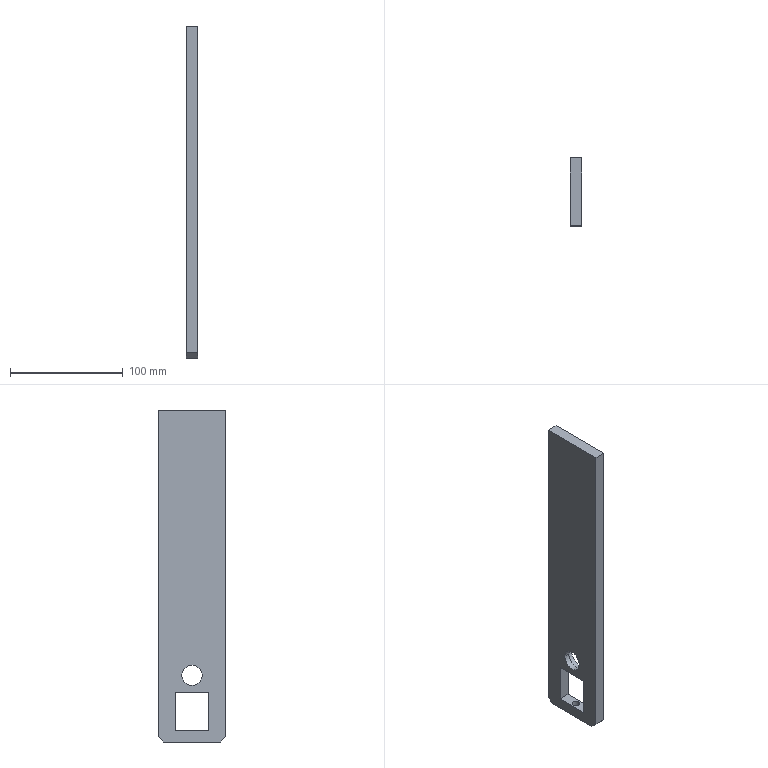Component | SolidWorks | SupportPlate-2 | 1 solid | 25 faces | box 10 x 60 x 294 mm | volume 162382 mm3 | plane 15 | cylinder 10 | commonest cylinder face diameters 8 x4 6.8 x2 18 x2 21 x2
build123d program:
from build123d import *

# Parameters (mm, degrees)
SKETCH1_W             = 60
SKETCH1_H             = 300
BOSS_EXTRUDE1_DEPTH   = 10
SKETCH2_R             = 10.5
CUT_EXTRUDE1_DEPTH    = 5
SKETCH3_R             = 9
CUT_EXTRUDE2_DEPTH    = 306.982
SKETCH4_W             = 30
SKETCH4_H             = 50
CUT_EXTRUDE3_DEPTH    = 307.105
SKETCH5_R             = 4
CUT_EXTRUDE4_DEPTH    = 2
SKETCH6_W             = 30
SKETCH6_H             = 16
BOSS_EXTRUDE2_DEPTH   = 10
SKETCH7_W             = 74.928
SKETCH7_H             = 16.817
CUT_EXTRUDE5_DEPTH    = 307.105
CHAMFER1_SIZE         = 5
M8_TAPPED_HOLE1_D     = 6.8
M8_TAPPED_HOLE1_DEPTH = 19.75
M8_TAPPED_HOLE1_TIP   = 2.043


with BuildPart() as part:
    # Sketch1 → Boss-Extrude1 (new body)
    with BuildSketch(Plane.XY):
        with Locations((30, -150)):
            Rectangle(SKETCH1_W, SKETCH1_H)
    extrude(amount=BOSS_EXTRUDE1_DEPTH)

    # Sketch2 → Cut-Extrude1 (cut)
    with BuildSketch(Plane.XY.offset(10)):
        with Locations((30, -25)):
            Circle(SKETCH2_R)
        with Locations((30, -65)):
            Circle(SKETCH2_R)
    extrude(amount=-CUT_EXTRUDE1_DEPTH, mode=Mode.SUBTRACT)

    # Sketch3 → Cut-Extrude2 (cut, through all)
    with BuildSketch(Plane.XY.offset(5)):
        with Locations((30, -25)):
            Circle(SKETCH3_R)
        with Locations((30, -65)):
            Circle(SKETCH3_R)
    extrude(amount=-CUT_EXTRUDE2_DEPTH, mode=Mode.SUBTRACT)

    # Sketch4 → Cut-Extrude3 (cut, through all)
    with BuildSketch(Plane.XY.offset(10)):
        with Locations((30, -25)):
            Rectangle(SKETCH4_W, SKETCH4_H)
    extrude(amount=-CUT_EXTRUDE3_DEPTH, mode=Mode.SUBTRACT)

    # Sketch5 → Cut-Extrude4 (cut)
    with BuildSketch(Plane(origin=(0, -50, 0), x_dir=(1, 0, 0), z_dir=(0, 1, 0))):
        with Locations(Location((19.5, -5, 0), (0, 0, 270))):
            Circle(SKETCH5_R)
        with Locations(Location((40.5, -5, 0), (0, 0, 270))):
            Circle(SKETCH5_R)
    extrude(amount=-CUT_EXTRUDE4_DEPTH, mode=Mode.SUBTRACT)

    # Sketch6 → Boss-Extrude2 (add)
    with BuildSketch(Plane(origin=(0, 0, 0), x_dir=(-1, 0, 0), z_dir=(0, 0, -1))):
        with Locations((-30, -8)):
            Rectangle(SKETCH6_W, SKETCH6_H)
    extrude(amount=-BOSS_EXTRUDE2_DEPTH)

    # Sketch7 → Cut-Extrude5 (cut, through all)
    with BuildSketch(Plane.XY.offset(10)):
        with Locations((27.689, 2.409)):
            Rectangle(SKETCH7_W, SKETCH7_H)
    extrude(amount=-CUT_EXTRUDE5_DEPTH, mode=Mode.SUBTRACT)

    # Chamfer1
    chamfer1_edges = [part.edges().sort_by_distance(p)[0] for p in [
        (0, -6, 5),
        (60, -6, 5),
    ]]
    chamfer(chamfer1_edges, length=CHAMFER1_SIZE)

    # M8 Tapped Hole1
    with Locations(Plane(origin=(0, -6, 0), x_dir=(1, 0, 0), z_dir=(0, 1, 0))):
        with Locations((30, -5)):
            Hole(M8_TAPPED_HOLE1_D / 2, depth=M8_TAPPED_HOLE1_DEPTH)
            with Locations((0, 0, -(M8_TAPPED_HOLE1_DEPTH + M8_TAPPED_HOLE1_TIP / 2))):  # 118° drill point
                Cone(0, M8_TAPPED_HOLE1_D / 2, M8_TAPPED_HOLE1_TIP, mode=Mode.SUBTRACT)


solid = part.part

# Placed as in the assembly
solid = solid.moved(Location((0, 0, -207.268), (-90, 90, 0)))
STEP:
#1=COLOUR_RGB('',0.7922,0.8196,0.9333);
#2=FILL_AREA_STYLE_COLOUR('',#1);
#3=FILL_AREA_STYLE('',(#2));
#4=SURFACE_STYLE_FILL_AREA(#3);
#5=SURFACE_SIDE_STYLE('',(#4));
#6=SURFACE_STYLE_USAGE(.BOTH.,#5);
#7=PRESENTATION_STYLE_ASSIGNMENT((#6));
#8=CARTESIAN_POINT('',(0.3307,-1.181,-7.53));
#9=VERTEX_POINT('',#8);
#10=CARTESIAN_POINT('',(0.06299,-1.181,-7.53));
#11=VERTEX_POINT('',#10);
#12=CARTESIAN_POINT('',(0.1969,-1.181,-7.53));
#13=DIRECTION('',(0.,0.,1.));
#14=DIRECTION('',(-1.,0.,0.));
#15=AXIS2_PLACEMENT_3D('',#12,#13,#14);
#16=CIRCLE('',#15,0.1339);
#17=EDGE_CURVE('',#9,#11,#16,.T.);
#18=ORIENTED_EDGE('',*,*,#17,.T.);
#19=CARTESIAN_POINT('',(0.06299,-1.181,-7.924));
#20=VERTEX_POINT('',#19);
#21=CARTESIAN_POINT('',(0.06299,-1.181,-7.924));
#22=DIRECTION('',(-0.,-0.,-1.));
#23=VECTOR('',#22,39.37);
#24=LINE('',#21,#23);
#25=EDGE_CURVE('',#11,#20,#24,.T.);
#26=ORIENTED_EDGE('',*,*,#25,.T.);
#27=CARTESIAN_POINT('',(0.3307,-1.181,-7.924));
#28=VERTEX_POINT('',#27);
#29=CARTESIAN_POINT('',(0.1969,-1.181,-7.924));
#30=DIRECTION('',(-0.,-0.,-1.));
#31=DIRECTION('',(1.,0.,0.));
#32=AXIS2_PLACEMENT_3D('',#29,#30,#31);
#33=CIRCLE('',#32,0.1339);
#34=EDGE_CURVE('',#20,#28,#33,.T.);
#35=ORIENTED_EDGE('',*,*,#34,.T.);
#36=CARTESIAN_POINT('',(0.3307,-1.181,-7.924));
#37=DIRECTION('',(-0.,-0.,-1.));
#38=VECTOR('',#37,39.37);
#39=LINE('',#36,#38);
#40=EDGE_CURVE('',#9,#28,#39,.T.);
#41=ORIENTED_EDGE('',*,*,#40,.F.);
#42=EDGE_LOOP('',(#18,#26,#35,#41));
#43=FACE_OUTER_BOUND('',#42,.T.);
#44=CARTESIAN_POINT('',(0.1969,-1.181,-7.924));
#45=DIRECTION('',(-0.,-0.,-1.));
#46=DIRECTION('',(1.,0.,0.));
#47=AXIS2_PLACEMENT_3D('',#44,#45,#46);
#48=CYLINDRICAL_SURFACE('',#47,0.1339);
#49=ADVANCED_FACE('',(#43),#48,.F.);
#50=CARTESIAN_POINT('',(0.03937,-1.594,-6.113));
#51=VERTEX_POINT('',#50);
#52=CARTESIAN_POINT('',(0.3543,-1.594,-6.113));
#53=VERTEX_POINT('',#52);
#54=CARTESIAN_POINT('',(0.1969,-1.594,-6.113));
#55=DIRECTION('',(-0.,-0.,-1.));
#56=DIRECTION('',(1.,0.,0.));
#57=AXIS2_PLACEMENT_3D('',#54,#55,#56);
#58=CIRCLE('',#57,0.1575);
#59=EDGE_CURVE('',#51,#53,#58,.T.);
#60=ORIENTED_EDGE('',*,*,#59,.F.);
#61=CARTESIAN_POINT('',(0.03937,-1.594,-6.192));
#62=VERTEX_POINT('',#61);
#63=CARTESIAN_POINT('',(0.03937,-1.594,-6.113));
#64=DIRECTION('',(-0.,-0.,-1.));
#65=VECTOR('',#64,39.37);
#66=LINE('',#63,#65);
#67=EDGE_CURVE('',#51,#62,#66,.T.);
#68=ORIENTED_EDGE('',*,*,#67,.T.);
#69=CARTESIAN_POINT('',(0.3543,-1.594,-6.192));
#70=VERTEX_POINT('',#69);
#71=CARTESIAN_POINT('',(0.1969,-1.594,-6.192));
#72=DIRECTION('',(-0.,-0.,-1.));
#73=DIRECTION('',(1.,0.,0.));
#74=AXIS2_PLACEMENT_3D('',#71,#72,#73);
#75=CIRCLE('',#74,0.1575);
#76=EDGE_CURVE('',#62,#70,#75,.T.);
#77=ORIENTED_EDGE('',*,*,#76,.T.);
#78=CARTESIAN_POINT('',(0.3543,-1.594,-6.113));
#79=DIRECTION('',(-0.,-0.,-1.));
#80=VECTOR('',#79,39.37);
#81=LINE('',#78,#80);
#82=EDGE_CURVE('',#53,#70,#81,.T.);
#83=ORIENTED_EDGE('',*,*,#82,.F.);
#84=EDGE_LOOP('',(#60,#68,#77,#83));
#85=FACE_OUTER_BOUND('',#84,.T.);
#86=CARTESIAN_POINT('',(0.1969,-1.594,-6.113));
#87=DIRECTION('',(-0.,-0.,-1.));
#88=DIRECTION('',(1.,0.,0.));
#89=AXIS2_PLACEMENT_3D('',#86,#87,#88);
#90=CYLINDRICAL_SURFACE('',#89,0.1575);
#91=ADVANCED_FACE('',(#85),#90,.F.);
#92=CARTESIAN_POINT('',(0.03937,-0.7677,-6.113));
#93=VERTEX_POINT('',#92);
#94=CARTESIAN_POINT('',(0.3543,-0.7677,-6.113));
#95=VERTEX_POINT('',#94);
#96=CARTESIAN_POINT('',(0.1969,-0.7677,-6.113));
#97=DIRECTION('',(-0.,-0.,-1.));
#98=DIRECTION('',(1.,0.,0.));
#99=AXIS2_PLACEMENT_3D('',#96,#97,#98);
#100=CIRCLE('',#99,0.1575);
#101=EDGE_CURVE('',#93,#95,#100,.T.);
#102=ORIENTED_EDGE('',*,*,#101,.F.);
#103=CARTESIAN_POINT('',(0.03937,-0.7677,-6.192));
#104=VERTEX_POINT('',#103);
#105=CARTESIAN_POINT('',(0.03937,-0.7677,-6.113));
#106=DIRECTION('',(-0.,-0.,-1.));
#107=VECTOR('',#106,39.37);
#108=LINE('',#105,#107);
#109=EDGE_CURVE('',#93,#104,#108,.T.);
#110=ORIENTED_EDGE('',*,*,#109,.T.);
#111=CARTESIAN_POINT('',(0.3543,-0.7677,-6.192));
#112=VERTEX_POINT('',#111);
#113=CARTESIAN_POINT('',(0.1969,-0.7677,-6.192));
#114=DIRECTION('',(-0.,-0.,-1.));
#115=DIRECTION('',(1.,0.,0.));
#116=AXIS2_PLACEMENT_3D('',#113,#114,#115);
#117=CIRCLE('',#116,0.1575);
#118=EDGE_CURVE('',#104,#112,#117,.T.);
#119=ORIENTED_EDGE('',*,*,#118,.T.);
#120=CARTESIAN_POINT('',(0.3543,-0.7677,-6.113));
#121=DIRECTION('',(-0.,-0.,-1.));
#122=VECTOR('',#121,39.37);
#123=LINE('',#120,#122);
#124=EDGE_CURVE('',#95,#112,#123,.T.);
#125=ORIENTED_EDGE('',*,*,#124,.F.);
#126=EDGE_LOOP('',(#102,#110,#119,#125));
#127=FACE_OUTER_BOUND('',#126,.T.);
#128=CARTESIAN_POINT('',(0.1969,-0.7677,-6.113));
#129=DIRECTION('',(-0.,-0.,-1.));
#130=DIRECTION('',(1.,0.,0.));
#131=AXIS2_PLACEMENT_3D('',#128,#129,#130);
#132=CYLINDRICAL_SURFACE('',#131,0.1575);
#133=ADVANCED_FACE('',(#127),#132,.F.);
#134=CARTESIAN_POINT('',(-0.,-0.8268,-5.601));
#135=VERTEX_POINT('',#134);
#136=CARTESIAN_POINT('',(-0.,-1.535,-5.601));
#137=VERTEX_POINT('',#136);
#138=CARTESIAN_POINT('',(-0.,-1.181,-5.601));
#139=DIRECTION('',(1.,0.,-0.));
#140=DIRECTION('',(0.,-1.,0.));
#141=AXIS2_PLACEMENT_3D('',#138,#139,#140);
#142=CIRCLE('',#141,0.3543);
#143=EDGE_CURVE('',#135,#137,#142,.T.);
#144=ORIENTED_EDGE('',*,*,#143,.F.);
#145=CARTESIAN_POINT('',(0.1969,-0.8268,-5.601));
#146=VERTEX_POINT('',#145);
#147=CARTESIAN_POINT('',(-0.,-0.8268,-5.601));
#148=DIRECTION('',(1.,0.,-0.));
#149=VECTOR('',#148,39.37);
#150=LINE('',#147,#149);
#151=EDGE_CURVE('',#135,#146,#150,.T.);
#152=ORIENTED_EDGE('',*,*,#151,.T.);
#153=CARTESIAN_POINT('',(0.1969,-1.535,-5.601));
#154=VERTEX_POINT('',#153);
#155=CARTESIAN_POINT('',(0.1969,-1.181,-5.601));
#156=DIRECTION('',(1.,0.,-0.));
#157=DIRECTION('',(0.,-1.,0.));
#158=AXIS2_PLACEMENT_3D('',#155,#156,#157);
#159=CIRCLE('',#158,0.3543);
#160=EDGE_CURVE('',#146,#154,#159,.T.);
#161=ORIENTED_EDGE('',*,*,#160,.T.);
#162=CARTESIAN_POINT('',(-0.,-1.535,-5.601));
#163=DIRECTION('',(1.,0.,-0.));
#164=VECTOR('',#163,39.37);
#165=LINE('',#162,#164);
#166=EDGE_CURVE('',#137,#154,#165,.T.);
#167=ORIENTED_EDGE('',*,*,#166,.F.);
#168=EDGE_LOOP('',(#144,#152,#161,#167));
#169=FACE_OUTER_BOUND('',#168,.T.);
#170=CARTESIAN_POINT('',(-0.,-1.181,-5.601));
#171=DIRECTION('',(1.,0.,-0.));
#172=DIRECTION('',(0.,-1.,0.));
#173=AXIS2_PLACEMENT_3D('',#170,#171,#172);
#174=CYLINDRICAL_SURFACE('',#173,0.3543);
#175=ADVANCED_FACE('',(#169),#174,.F.);
#176=CARTESIAN_POINT('',(0.1969,-0.7677,-5.601));
#177=VERTEX_POINT('',#176);
#178=CARTESIAN_POINT('',(0.1969,-1.594,-5.601));
#179=VERTEX_POINT('',#178);
#180=CARTESIAN_POINT('',(0.1969,-1.181,-5.601));
#181=DIRECTION('',(1.,0.,-0.));
#182=DIRECTION('',(0.,-1.,0.));
#183=AXIS2_PLACEMENT_3D('',#180,#181,#182);
#184=CIRCLE('',#183,0.4134);
#185=EDGE_CURVE('',#177,#179,#184,.T.);
#186=ORIENTED_EDGE('',*,*,#185,.F.);
#187=CARTESIAN_POINT('',(0.3937,-0.7677,-5.601));
#188=VERTEX_POINT('',#187);
#189=CARTESIAN_POINT('',(0.1969,-0.7677,-5.601));
#190=DIRECTION('',(1.,0.,-0.));
#191=VECTOR('',#190,39.37);
#192=LINE('',#189,#191);
#193=EDGE_CURVE('',#177,#188,#192,.T.);
#194=ORIENTED_EDGE('',*,*,#193,.T.);
#195=CARTESIAN_POINT('',(0.3937,-1.594,-5.601));
#196=VERTEX_POINT('',#195);
#197=CARTESIAN_POINT('',(0.3937,-1.181,-5.601));
#198=DIRECTION('',(1.,0.,-0.));
#199=DIRECTION('',(0.,-1.,0.));
#200=AXIS2_PLACEMENT_3D('',#197,#198,#199);
#201=CIRCLE('',#200,0.4134);
#202=EDGE_CURVE('',#188,#196,#201,.T.);
#203=ORIENTED_EDGE('',*,*,#202,.T.);
#204=CARTESIAN_POINT('',(0.1969,-1.594,-5.601));
#205=DIRECTION('',(1.,0.,-0.));
#206=VECTOR('',#205,39.37);
#207=LINE('',#204,#206);
#208=EDGE_CURVE('',#179,#196,#207,.T.);
#209=ORIENTED_EDGE('',*,*,#208,.F.);
#210=EDGE_LOOP('',(#186,#194,#203,#209));
#211=FACE_OUTER_BOUND('',#210,.T.);
#212=CARTESIAN_POINT('',(0.1969,-1.181,-5.601));
#213=DIRECTION('',(1.,0.,-0.));
#214=DIRECTION('',(0.,-1.,0.));
#215=AXIS2_PLACEMENT_3D('',#212,#213,#214);
#216=CYLINDRICAL_SURFACE('',#215,0.4134);
#217=ADVANCED_FACE('',(#211),#216,.F.);
#218=CARTESIAN_POINT('',(0.3937,-0.,-7.727));
#219=VERTEX_POINT('',#218);
#220=CARTESIAN_POINT('',(0.3937,-0.,3.651));
#221=VERTEX_POINT('',#220);
#222=CARTESIAN_POINT('',(0.3937,0.,-8.16));
#223=DIRECTION('',(0.,-0.,1.));
#224=VECTOR('',#223,39.37);
#225=LINE('',#222,#224);
#226=EDGE_CURVE('',#219,#221,#225,.T.);
#227=ORIENTED_EDGE('',*,*,#226,.F.);
#228=CARTESIAN_POINT('',(-0.,-0.,-7.727));
#229=VERTEX_POINT('',#228);
#230=CARTESIAN_POINT('',(0.3937,-0.,-7.727));
#231=DIRECTION('',(-1.,-0.,0.));
#232=VECTOR('',#231,39.37);
#233=LINE('',#230,#232);
#234=EDGE_CURVE('',#219,#229,#233,.T.);
#235=ORIENTED_EDGE('',*,*,#234,.T.);
#236=CARTESIAN_POINT('',(-0.,-0.,3.651));
#237=VERTEX_POINT('',#236);
#238=CARTESIAN_POINT('',(-0.,0.,-8.16));
#239=DIRECTION('',(0.,-0.,1.));
#240=VECTOR('',#239,39.37);
#241=LINE('',#238,#240);
#242=EDGE_CURVE('',#229,#237,#241,.T.);
#243=ORIENTED_EDGE('',*,*,#242,.T.);
#244=CARTESIAN_POINT('',(0.3937,-0.,3.651));
#245=DIRECTION('',(-1.,-0.,0.));
#246=VECTOR('',#245,39.37);
#247=LINE('',#244,#246);
#248=EDGE_CURVE('',#221,#237,#247,.T.);
#249=ORIENTED_EDGE('',*,*,#248,.F.);
#250=EDGE_LOOP('',(#227,#235,#243,#249));
#251=FACE_OUTER_BOUND('',#250,.T.);
#252=CARTESIAN_POINT('',(0.3937,0.,-8.16));
#253=DIRECTION('',(0.,-1.,-0.));
#254=DIRECTION('',(-0.,0.,-1.));
#255=AXIS2_PLACEMENT_3D('',#252,#253,#254);
#256=PLANE('',#255);
#257=ADVANCED_FACE('',(#251),#256,.F.);
#258=CARTESIAN_POINT('',(-0.,-2.362,3.651));
#259=VERTEX_POINT('',#258);
#260=CARTESIAN_POINT('',(-0.,-0.,3.651));
#261=DIRECTION('',(0.,-1.,0.));
#262=VECTOR('',#261,39.37);
#263=LINE('',#260,#262);
#264=EDGE_CURVE('',#237,#259,#263,.T.);
#265=ORIENTED_EDGE('',*,*,#264,.T.);
#266=CARTESIAN_POINT('',(0.3937,-2.362,3.651));
#267=VERTEX_POINT('',#266);
#268=CARTESIAN_POINT('',(0.3937,-2.362,3.651));
#269=DIRECTION('',(-1.,-0.,0.));
#270=VECTOR('',#269,39.37);
#271=LINE('',#268,#270);
#272=EDGE_CURVE('',#267,#259,#271,.T.);
#273=ORIENTED_EDGE('',*,*,#272,.F.);
#274=CARTESIAN_POINT('',(0.3937,-0.,3.651));
#275=DIRECTION('',(0.,-1.,0.));
#276=VECTOR('',#275,39.37);
#277=LINE('',#274,#276);
#278=EDGE_CURVE('',#221,#267,#277,.T.);
#279=ORIENTED_EDGE('',*,*,#278,.F.);
#280=ORIENTED_EDGE('',*,*,#248,.T.);
#281=EDGE_LOOP('',(#265,#273,#279,#280));
#282=FACE_OUTER_BOUND('',#281,.T.);
#283=CARTESIAN_POINT('',(0.3937,-0.,3.651));
#284=DIRECTION('',(-0.,-0.,-1.));
#285=DIRECTION('',(1.,0.,-0.));
#286=AXIS2_PLACEMENT_3D('',#283,#284,#285);
#287=PLANE('',#286);
#288=ADVANCED_FACE('',(#282),#287,.F.);
#289=CARTESIAN_POINT('',(-0.,-2.362,-7.727));
#290=VERTEX_POINT('',#289);
#291=CARTESIAN_POINT('',(-0.,-2.362,-8.16));
#292=DIRECTION('',(-0.,0.,-1.));
#293=VECTOR('',#292,39.37);
#294=LINE('',#291,#293);
#295=EDGE_CURVE('',#259,#290,#294,.T.);
#296=ORIENTED_EDGE('',*,*,#295,.T.);
#297=CARTESIAN_POINT('',(0.3937,-2.362,-7.727));
#298=VERTEX_POINT('',#297);
#299=CARTESIAN_POINT('',(0.3937,-2.362,-7.727));
#300=DIRECTION('',(1.,0.,-0.));
#301=VECTOR('',#300,39.37);
#302=LINE('',#299,#301);
#303=EDGE_CURVE('',#290,#298,#302,.T.);
#304=ORIENTED_EDGE('',*,*,#303,.T.);
#305=CARTESIAN_POINT('',(0.3937,-2.362,-8.16));
#306=DIRECTION('',(-0.,0.,-1.));
#307=VECTOR('',#306,39.37);
#308=LINE('',#305,#307);
#309=EDGE_CURVE('',#267,#298,#308,.T.);
#310=ORIENTED_EDGE('',*,*,#309,.F.);
#311=ORIENTED_EDGE('',*,*,#272,.T.);
#312=EDGE_LOOP('',(#296,#304,#310,#311));
#313=FACE_OUTER_BOUND('',#312,.T.);
#314=CARTESIAN_POINT('',(0.3937,-2.362,-8.16));
#315=DIRECTION('',(-0.,1.,0.));
#316=DIRECTION('',(0.,-0.,1.));
#317=AXIS2_PLACEMENT_3D('',#314,#315,#316);
#318=PLANE('',#317);
#319=ADVANCED_FACE('',(#313),#318,.F.);
#320=CARTESIAN_POINT('',(0.3937,-0.1969,-7.924));
#321=VERTEX_POINT('',#320);
#322=CARTESIAN_POINT('',(0.3937,-2.165,-7.924));
#323=VERTEX_POINT('',#322);
#324=CARTESIAN_POINT('',(0.3937,0.3848,-7.924));
#325=DIRECTION('',(0.,-1.,0.));
#326=VECTOR('',#325,39.37);
#327=LINE('',#324,#326);
#328=EDGE_CURVE('',#321,#323,#327,.T.);
#329=ORIENTED_EDGE('',*,*,#328,.F.);
#330=CARTESIAN_POINT('',(0.3937,-0.2165,-7.944));
#331=DIRECTION('',(0.,0.7071,0.7071));
#332=VECTOR('',#331,39.37);
#333=LINE('',#330,#332);
#334=EDGE_CURVE('',#321,#219,#333,.T.);
#335=ORIENTED_EDGE('',*,*,#334,.T.);
#336=ORIENTED_EDGE('',*,*,#226,.T.);
#337=ORIENTED_EDGE('',*,*,#278,.T.);
#338=ORIENTED_EDGE('',*,*,#309,.T.);
#339=CARTESIAN_POINT('',(0.3937,-0.9646,-9.125));
#340=DIRECTION('',(-0.,0.7071,-0.7071));
#341=VECTOR('',#340,39.37);
#342=LINE('',#339,#341);
#343=EDGE_CURVE('',#298,#323,#342,.T.);
#344=ORIENTED_EDGE('',*,*,#343,.T.);
#345=EDGE_LOOP('',(#329,#335,#336,#337,#338,#344));
#346=FACE_OUTER_BOUND('',#345,.T.);
#347=CARTESIAN_POINT('',(0.3937,-0.5906,-7.53));
#348=VERTEX_POINT('',#347);
#349=CARTESIAN_POINT('',(0.3937,-0.5906,-6.192));
#350=VERTEX_POINT('',#349);
#351=CARTESIAN_POINT('',(0.3937,-0.5906,-8.16));
#352=DIRECTION('',(0.,0.,1.));
#353=VECTOR('',#352,39.37);
#354=LINE('',#351,#353);
#355=EDGE_CURVE('',#348,#350,#354,.T.);
#356=ORIENTED_EDGE('',*,*,#355,.F.);
#357=CARTESIAN_POINT('',(0.3937,-1.772,-7.53));
#358=VERTEX_POINT('',#357);
#359=CARTESIAN_POINT('',(0.3937,-1.772,-7.53));
#360=DIRECTION('',(-0.,1.,-0.));
#361=VECTOR('',#360,39.37);
#362=LINE('',#359,#361);
#363=EDGE_CURVE('',#358,#348,#362,.T.);
#364=ORIENTED_EDGE('',*,*,#363,.F.);
#365=CARTESIAN_POINT('',(0.3937,-1.772,-6.192));
#366=VERTEX_POINT('',#365);
#367=CARTESIAN_POINT('',(0.3937,-1.772,-8.16));
#368=DIRECTION('',(-0.,-0.,-1.));
#369=VECTOR('',#368,39.37);
#370=LINE('',#367,#369);
#371=EDGE_CURVE('',#366,#358,#370,.T.);
#372=ORIENTED_EDGE('',*,*,#371,.F.);
#373=CARTESIAN_POINT('',(0.3937,-0.5906,-6.192));
#374=DIRECTION('',(0.,-1.,0.));
#375=VECTOR('',#374,39.37);
#376=LINE('',#373,#375);
#377=EDGE_CURVE('',#350,#366,#376,.T.);
#378=ORIENTED_EDGE('',*,*,#377,.F.);
#379=EDGE_LOOP('',(#356,#364,#372,#378));
#380=FACE_BOUND('',#379,.T.);
#381=CARTESIAN_POINT('',(0.3937,-1.181,-5.601));
#382=DIRECTION('',(1.,0.,-0.));
#383=DIRECTION('',(0.,-1.,0.));
#384=AXIS2_PLACEMENT_3D('',#381,#382,#383);
#385=CIRCLE('',#384,0.4134);
#386=EDGE_CURVE('',#196,#188,#385,.T.);
#387=ORIENTED_EDGE('',*,*,#386,.F.);
#388=ORIENTED_EDGE('',*,*,#202,.F.);
#389=EDGE_LOOP('',(#387,#388));
#390=FACE_BOUND('',#389,.T.);
#391=CARTESIAN_POINT('',(0.3937,0.,-8.16));
#392=DIRECTION('',(1.,0.,-0.));
#393=DIRECTION('',(0.,-1.,0.));
#394=AXIS2_PLACEMENT_3D('',#391,#392,#393);
#395=PLANE('',#394);
#396=ADVANCED_FACE('',(#346,#380,#390),#395,.T.);
#397=CARTESIAN_POINT('',(-0.,-1.772,-7.53));
#398=VERTEX_POINT('',#397);
#399=CARTESIAN_POINT('',(-0.,-0.5906,-7.53));
#400=VERTEX_POINT('',#399);
#401=CARTESIAN_POINT('',(-0.,-1.772,-7.53));
#402=DIRECTION('',(-0.,1.,-0.));
#403=VECTOR('',#402,39.37);
#404=LINE('',#401,#403);
#405=EDGE_CURVE('',#398,#400,#404,.T.);
#406=ORIENTED_EDGE('',*,*,#405,.T.);
#407=CARTESIAN_POINT('',(-0.,-0.5906,-6.192));
#408=VERTEX_POINT('',#407);
#409=CARTESIAN_POINT('',(-0.,-0.5906,-8.16));
#410=DIRECTION('',(0.,0.,1.));
#411=VECTOR('',#410,39.37);
#412=LINE('',#409,#411);
#413=EDGE_CURVE('',#400,#408,#412,.T.);
#414=ORIENTED_EDGE('',*,*,#413,.T.);
#415=CARTESIAN_POINT('',(-0.,-1.772,-6.192));
#416=VERTEX_POINT('',#415);
#417=CARTESIAN_POINT('',(-0.,-0.5906,-6.192));
#418=DIRECTION('',(0.,-1.,0.));
#419=VECTOR('',#418,39.37);
#420=LINE('',#417,#419);
#421=EDGE_CURVE('',#408,#416,#420,.T.);
#422=ORIENTED_EDGE('',*,*,#421,.T.);
#423=CARTESIAN_POINT('',(-0.,-1.772,-8.16));
#424=DIRECTION('',(-0.,-0.,-1.));
#425=VECTOR('',#424,39.37);
#426=LINE('',#423,#425);
#427=EDGE_CURVE('',#416,#398,#426,.T.);
#428=ORIENTED_EDGE('',*,*,#427,.T.);
#429=EDGE_LOOP('',(#406,#414,#422,#428));
#430=FACE_BOUND('',#429,.T.);
#431=ORIENTED_EDGE('',*,*,#242,.F.);
#432=CARTESIAN_POINT('',(-0.,-0.1969,-7.924));
#433=VERTEX_POINT('',#432);
#434=CARTESIAN_POINT('',(-0.,-0.,-7.727));
#435=DIRECTION('',(-0.,-0.7071,-0.7071));
#436=VECTOR('',#435,39.37);
#437=LINE('',#434,#436);
#438=EDGE_CURVE('',#229,#433,#437,.T.);
#439=ORIENTED_EDGE('',*,*,#438,.T.);
#440=CARTESIAN_POINT('',(-0.,-2.165,-7.924));
#441=VERTEX_POINT('',#440);
#442=CARTESIAN_POINT('',(-0.,0.,-7.924));
#443=DIRECTION('',(0.,-1.,0.));
#444=VECTOR('',#443,39.37);
#445=LINE('',#442,#444);
#446=EDGE_CURVE('',#433,#441,#445,.T.);
#447=ORIENTED_EDGE('',*,*,#446,.T.);
#448=CARTESIAN_POINT('',(-0.,-2.362,-7.727));
#449=DIRECTION('',(0.,-0.7071,0.7071));
#450=VECTOR('',#449,39.37);
#451=LINE('',#448,#450);
#452=EDGE_CURVE('',#441,#290,#451,.T.);
#453=ORIENTED_EDGE('',*,*,#452,.T.);
#454=ORIENTED_EDGE('',*,*,#295,.F.);
#455=ORIENTED_EDGE('',*,*,#264,.F.);
#456=EDGE_LOOP('',(#431,#439,#447,#453,#454,#455));
#457=FACE_OUTER_BOUND('',#456,.T.);
#458=CARTESIAN_POINT('',(-0.,-1.181,-5.601));
#459=DIRECTION('',(1.,0.,-0.));
#460=DIRECTION('',(0.,-1.,0.));
#461=AXIS2_PLACEMENT_3D('',#458,#459,#460);
#462=CIRCLE('',#461,0.3543);
#463=EDGE_CURVE('',#137,#135,#462,.T.);
#464=ORIENTED_EDGE('',*,*,#463,.T.);
#465=ORIENTED_EDGE('',*,*,#143,.T.);
#466=EDGE_LOOP('',(#464,#465));
#467=FACE_BOUND('',#466,.T.);
#468=CARTESIAN_POINT('',(-0.,0.,-8.16));
#469=DIRECTION('',(1.,0.,-0.));
#470=DIRECTION('',(0.,-1.,0.));
#471=AXIS2_PLACEMENT_3D('',#468,#469,#470);
#472=PLANE('',#471);
#473=ADVANCED_FACE('',(#430,#457,#467),#472,.F.);
#474=ORIENTED_EDGE('',*,*,#193,.F.);
#475=CARTESIAN_POINT('',(0.1969,-1.181,-5.601));
#476=DIRECTION('',(1.,0.,-0.));
#477=DIRECTION('',(0.,-1.,0.));
#478=AXIS2_PLACEMENT_3D('',#475,#476,#477);
#479=CIRCLE('',#478,0.4134);
#480=EDGE_CURVE('',#179,#177,#479,.T.);
#481=ORIENTED_EDGE('',*,*,#480,.F.);
#482=ORIENTED_EDGE('',*,*,#208,.T.);
#483=ORIENTED_EDGE('',*,*,#386,.T.);
#484=EDGE_LOOP('',(#474,#481,#482,#483));
#485=FACE_OUTER_BOUND('',#484,.T.);
#486=CARTESIAN_POINT('',(0.1969,-1.181,-5.601));
#487=DIRECTION('',(1.,0.,-0.));
#488=DIRECTION('',(0.,-1.,0.));
#489=AXIS2_PLACEMENT_3D('',#486,#487,#488);
#490=CYLINDRICAL_SURFACE('',#489,0.4134);
#491=ADVANCED_FACE('',(#485),#490,.F.);
#492=CARTESIAN_POINT('',(0.1969,-1.181,-5.601));
#493=DIRECTION('',(1.,0.,-0.));
#494=DIRECTION('',(0.,-1.,0.));
#495=AXIS2_PLACEMENT_3D('',#492,#493,#494);
#496=CIRCLE('',#495,0.3543);
#497=EDGE_CURVE('',#154,#146,#496,.T.);
#498=ORIENTED_EDGE('',*,*,#497,.F.);
#499=ORIENTED_EDGE('',*,*,#160,.F.);
#500=EDGE_LOOP('',(#498,#499));
#501=FACE_BOUND('',#500,.T.);
#502=ORIENTED_EDGE('',*,*,#480,.T.);
#503=ORIENTED_EDGE('',*,*,#185,.T.);
#504=EDGE_LOOP('',(#502,#503));
#505=FACE_OUTER_BOUND('',#504,.T.);
#506=CARTESIAN_POINT('',(0.1969,-1.181,-5.601));
#507=DIRECTION('',(1.,0.,-0.));
#508=DIRECTION('',(0.,-1.,0.));
#509=AXIS2_PLACEMENT_3D('',#506,#507,#508);
#510=PLANE('',#509);
#511=ADVANCED_FACE('',(#501,#505),#510,.T.);
#512=ORIENTED_EDGE('',*,*,#151,.F.);
#513=ORIENTED_EDGE('',*,*,#463,.F.);
#514=ORIENTED_EDGE('',*,*,#166,.T.);
#515=ORIENTED_EDGE('',*,*,#497,.T.);
#516=EDGE_LOOP('',(#512,#513,#514,#515));
#517=FACE_OUTER_BOUND('',#516,.T.);
#518=CARTESIAN_POINT('',(-0.,-1.181,-5.601));
#519=DIRECTION('',(1.,0.,-0.));
#520=DIRECTION('',(0.,-1.,0.));
#521=AXIS2_PLACEMENT_3D('',#518,#519,#520);
#522=CYLINDRICAL_SURFACE('',#521,0.3543);
#523=ADVANCED_FACE('',(#517),#522,.F.);
#524=ORIENTED_EDGE('',*,*,#413,.F.);
#525=CARTESIAN_POINT('',(1.732,-0.5906,-7.53));
#526=DIRECTION('',(-1.,-0.,0.));
#527=VECTOR('',#526,39.37);
#528=LINE('',#525,#527);
#529=EDGE_CURVE('',#348,#400,#528,.T.);
#530=ORIENTED_EDGE('',*,*,#529,.F.);
#531=ORIENTED_EDGE('',*,*,#355,.T.);
#532=CARTESIAN_POINT('',(-0.,-0.5906,-6.192));
#533=DIRECTION('',(1.,0.,-0.));
#534=VECTOR('',#533,39.37);
#535=LINE('',#532,#534);
#536=EDGE_CURVE('',#408,#350,#535,.T.);
#537=ORIENTED_EDGE('',*,*,#536,.F.);
#538=EDGE_LOOP('',(#524,#530,#531,#537));
#539=FACE_OUTER_BOUND('',#538,.T.);
#540=CARTESIAN_POINT('',(-0.,-0.5906,-8.16));
#541=DIRECTION('',(-0.,1.,-0.));
#542=DIRECTION('',(0.,0.,1.));
#543=AXIS2_PLACEMENT_3D('',#540,#541,#542);
#544=PLANE('',#543);
#545=ADVANCED_FACE('',(#539),#544,.F.);
#546=ORIENTED_EDGE('',*,*,#371,.T.);
#547=CARTESIAN_POINT('',(1.732,-1.772,-7.53));
#548=DIRECTION('',(-1.,-0.,0.));
#549=VECTOR('',#548,39.37);
#550=LINE('',#547,#549);
#551=EDGE_CURVE('',#358,#398,#550,.T.);
#552=ORIENTED_EDGE('',*,*,#551,.T.);
#553=ORIENTED_EDGE('',*,*,#427,.F.);
#554=CARTESIAN_POINT('',(-0.,-1.772,-6.192));
#555=DIRECTION('',(1.,0.,-0.));
#556=VECTOR('',#555,39.37);
#557=LINE('',#554,#556);
#558=EDGE_CURVE('',#416,#366,#557,.T.);
#559=ORIENTED_EDGE('',*,*,#558,.T.);
#560=EDGE_LOOP('',(#546,#552,#553,#559));
#561=FACE_OUTER_BOUND('',#560,.T.);
#562=CARTESIAN_POINT('',(-0.,-1.772,-8.16));
#563=DIRECTION('',(0.,-1.,0.));
#564=DIRECTION('',(-0.,-0.,-1.));
#565=AXIS2_PLACEMENT_3D('',#562,#563,#564);
#566=PLANE('',#565);
#567=ADVANCED_FACE('',(#561),#566,.F.);
#568=CARTESIAN_POINT('',(0.1969,-1.594,-6.192));
#569=DIRECTION('',(-0.,-0.,-1.));
#570=DIRECTION('',(1.,0.,0.));
#571=AXIS2_PLACEMENT_3D('',#568,#569,#570);
#572=CIRCLE('',#571,0.1575);
#573=EDGE_CURVE('',#70,#62,#572,.T.);
#574=ORIENTED_EDGE('',*,*,#573,.F.);
#575=ORIENTED_EDGE('',*,*,#76,.F.);
#576=EDGE_LOOP('',(#574,#575));
#577=FACE_BOUND('',#576,.T.);
#578=CARTESIAN_POINT('',(0.1969,-0.7677,-6.192));
#579=DIRECTION('',(-0.,-0.,-1.));
#580=DIRECTION('',(1.,0.,0.));
#581=AXIS2_PLACEMENT_3D('',#578,#579,#580);
#582=CIRCLE('',#581,0.1575);
#583=EDGE_CURVE('',#112,#104,#582,.T.);
#584=ORIENTED_EDGE('',*,*,#583,.F.);
#585=ORIENTED_EDGE('',*,*,#118,.F.);
#586=EDGE_LOOP('',(#584,#585));
#587=FACE_BOUND('',#586,.T.);
#588=ORIENTED_EDGE('',*,*,#377,.T.);
#589=ORIENTED_EDGE('',*,*,#558,.F.);
#590=ORIENTED_EDGE('',*,*,#421,.F.);
#591=ORIENTED_EDGE('',*,*,#536,.T.);
#592=EDGE_LOOP('',(#588,#589,#590,#591));
#593=FACE_OUTER_BOUND('',#592,.T.);
#594=CARTESIAN_POINT('',(-0.,-0.5906,-6.192));
#595=DIRECTION('',(0.,0.,1.));
#596=DIRECTION('',(-1.,-0.,0.));
#597=AXIS2_PLACEMENT_3D('',#594,#595,#596);
#598=PLANE('',#597);
#599=ADVANCED_FACE('',(#577,#587,#593),#598,.F.);
#600=ORIENTED_EDGE('',*,*,#109,.F.);
#601=CARTESIAN_POINT('',(0.1969,-0.7677,-6.113));
#602=DIRECTION('',(-0.,-0.,-1.));
#603=DIRECTION('',(1.,0.,0.));
#604=AXIS2_PLACEMENT_3D('',#601,#602,#603);
#605=CIRCLE('',#604,0.1575);
#606=EDGE_CURVE('',#95,#93,#605,.T.);
#607=ORIENTED_EDGE('',*,*,#606,.F.);
#608=ORIENTED_EDGE('',*,*,#124,.T.);
#609=ORIENTED_EDGE('',*,*,#583,.T.);
#610=EDGE_LOOP('',(#600,#607,#608,#609));
#611=FACE_OUTER_BOUND('',#610,.T.);
#612=CARTESIAN_POINT('',(0.1969,-0.7677,-6.113));
#613=DIRECTION('',(-0.,-0.,-1.));
#614=DIRECTION('',(1.,0.,0.));
#615=AXIS2_PLACEMENT_3D('',#612,#613,#614);
#616=CYLINDRICAL_SURFACE('',#615,0.1575);
#617=ADVANCED_FACE('',(#611),#616,.F.);
#618=ORIENTED_EDGE('',*,*,#606,.T.);
#619=ORIENTED_EDGE('',*,*,#101,.T.);
#620=EDGE_LOOP('',(#618,#619));
#621=FACE_OUTER_BOUND('',#620,.T.);
#622=CARTESIAN_POINT('',(0.1969,-0.7677,-6.113));
#623=DIRECTION('',(-0.,-0.,-1.));
#624=DIRECTION('',(1.,0.,-0.));
#625=AXIS2_PLACEMENT_3D('',#622,#623,#624);
#626=PLANE('',#625);
#627=ADVANCED_FACE('',(#621),#626,.T.);
#628=ORIENTED_EDGE('',*,*,#67,.F.);
#629=CARTESIAN_POINT('',(0.1969,-1.594,-6.113));
#630=DIRECTION('',(-0.,-0.,-1.));
#631=DIRECTION('',(1.,0.,0.));
#632=AXIS2_PLACEMENT_3D('',#629,#630,#631);
#633=CIRCLE('',#632,0.1575);
#634=EDGE_CURVE('',#53,#51,#633,.T.);
#635=ORIENTED_EDGE('',*,*,#634,.F.);
#636=ORIENTED_EDGE('',*,*,#82,.T.);
#637=ORIENTED_EDGE('',*,*,#573,.T.);
#638=EDGE_LOOP('',(#628,#635,#636,#637));
#639=FACE_OUTER_BOUND('',#638,.T.);
#640=CARTESIAN_POINT('',(0.1969,-1.594,-6.113));
#641=DIRECTION('',(-0.,-0.,-1.));
#642=DIRECTION('',(1.,0.,0.));
#643=AXIS2_PLACEMENT_3D('',#640,#641,#642);
#644=CYLINDRICAL_SURFACE('',#643,0.1575);
#645=ADVANCED_FACE('',(#639),#644,.F.);
#646=ORIENTED_EDGE('',*,*,#634,.T.);
#647=ORIENTED_EDGE('',*,*,#59,.T.);
#648=EDGE_LOOP('',(#646,#647));
#649=FACE_OUTER_BOUND('',#648,.T.);
#650=CARTESIAN_POINT('',(0.1969,-1.594,-6.113));
#651=DIRECTION('',(-0.,-0.,-1.));
#652=DIRECTION('',(1.,0.,-0.));
#653=AXIS2_PLACEMENT_3D('',#650,#651,#652);
#654=PLANE('',#653);
#655=ADVANCED_FACE('',(#649),#654,.T.);
#656=ORIENTED_EDGE('',*,*,#17,.F.);
#657=CARTESIAN_POINT('',(0.1969,-1.181,-7.53));
#658=DIRECTION('',(0.,0.,1.));
#659=DIRECTION('',(-1.,0.,0.));
#660=AXIS2_PLACEMENT_3D('',#657,#658,#659);
#661=CIRCLE('',#660,0.1339);
#662=EDGE_CURVE('',#11,#9,#661,.T.);
#663=ORIENTED_EDGE('',*,*,#662,.F.);
#664=EDGE_LOOP('',(#656,#663));
#665=FACE_BOUND('',#664,.T.);
#666=ORIENTED_EDGE('',*,*,#551,.F.);
#667=ORIENTED_EDGE('',*,*,#363,.T.);
#668=ORIENTED_EDGE('',*,*,#529,.T.);
#669=ORIENTED_EDGE('',*,*,#405,.F.);
#670=EDGE_LOOP('',(#666,#667,#668,#669));
#671=FACE_OUTER_BOUND('',#670,.T.);
#672=CARTESIAN_POINT('',(1.732,-1.772,-7.53));
#673=DIRECTION('',(0.,0.,1.));
#674=DIRECTION('',(-1.,-0.,0.));
#675=AXIS2_PLACEMENT_3D('',#672,#673,#674);
#676=PLANE('',#675);
#677=ADVANCED_FACE('',(#665,#671),#676,.T.);
#678=CARTESIAN_POINT('',(0.1969,-1.181,-7.924));
#679=DIRECTION('',(-0.,-0.,-1.));
#680=DIRECTION('',(1.,0.,0.));
#681=AXIS2_PLACEMENT_3D('',#678,#679,#680);
#682=CIRCLE('',#681,0.1339);
#683=EDGE_CURVE('',#28,#20,#682,.T.);
#684=ORIENTED_EDGE('',*,*,#683,.F.);
#685=ORIENTED_EDGE('',*,*,#34,.F.);
#686=EDGE_LOOP('',(#684,#685));
#687=FACE_BOUND('',#686,.T.);
#688=ORIENTED_EDGE('',*,*,#446,.F.);
#689=CARTESIAN_POINT('',(-0.,-0.1969,-7.924));
#690=DIRECTION('',(1.,0.,-0.));
#691=VECTOR('',#690,39.37);
#692=LINE('',#689,#691);
#693=EDGE_CURVE('',#433,#321,#692,.T.);
#694=ORIENTED_EDGE('',*,*,#693,.T.);
#695=ORIENTED_EDGE('',*,*,#328,.T.);
#696=CARTESIAN_POINT('',(-0.,-2.165,-7.924));
#697=DIRECTION('',(-1.,-0.,0.));
#698=VECTOR('',#697,39.37);
#699=LINE('',#696,#698);
#700=EDGE_CURVE('',#323,#441,#699,.T.);
#701=ORIENTED_EDGE('',*,*,#700,.T.);
#702=EDGE_LOOP('',(#688,#694,#695,#701));
#703=FACE_OUTER_BOUND('',#702,.T.);
#704=CARTESIAN_POINT('',(-0.,0.3848,-7.924));
#705=DIRECTION('',(0.,0.,1.));
#706=DIRECTION('',(-1.,-0.,0.));
#707=AXIS2_PLACEMENT_3D('',#704,#705,#706);
#708=PLANE('',#707);
#709=ADVANCED_FACE('',(#687,#703),#708,.F.);
#710=ORIENTED_EDGE('',*,*,#334,.F.);
#711=ORIENTED_EDGE('',*,*,#693,.F.);
#712=ORIENTED_EDGE('',*,*,#438,.F.);
#713=ORIENTED_EDGE('',*,*,#234,.F.);
#714=EDGE_LOOP('',(#710,#711,#712,#713));
#715=FACE_OUTER_BOUND('',#714,.T.);
#716=CARTESIAN_POINT('',(0.3937,-0.,-7.727));
#717=DIRECTION('',(0.,-0.7071,0.7071));
#718=DIRECTION('',(-1.,-0.,0.));
#719=AXIS2_PLACEMENT_3D('',#716,#717,#718);
#720=PLANE('',#719);
#721=ADVANCED_FACE('',(#715),#720,.F.);
#722=ORIENTED_EDGE('',*,*,#452,.F.);
#723=ORIENTED_EDGE('',*,*,#700,.F.);
#724=ORIENTED_EDGE('',*,*,#343,.F.);
#725=ORIENTED_EDGE('',*,*,#303,.F.);
#726=EDGE_LOOP('',(#722,#723,#724,#725));
#727=FACE_OUTER_BOUND('',#726,.T.);
#728=CARTESIAN_POINT('',(0.3937,-2.362,-7.727));
#729=DIRECTION('',(0.,0.7071,0.7071));
#730=DIRECTION('',(1.,0.,-0.));
#731=AXIS2_PLACEMENT_3D('',#728,#729,#730);
#732=PLANE('',#731);
#733=ADVANCED_FACE('',(#727),#732,.F.);
#734=ORIENTED_EDGE('',*,*,#25,.F.);
#735=ORIENTED_EDGE('',*,*,#662,.T.);
#736=ORIENTED_EDGE('',*,*,#40,.T.);
#737=ORIENTED_EDGE('',*,*,#683,.T.);
#738=EDGE_LOOP('',(#734,#735,#736,#737));
#739=FACE_OUTER_BOUND('',#738,.T.);
#740=CARTESIAN_POINT('',(0.1969,-1.181,-7.924));
#741=DIRECTION('',(-0.,-0.,-1.));
#742=DIRECTION('',(1.,0.,0.));
#743=AXIS2_PLACEMENT_3D('',#740,#741,#742);
#744=CYLINDRICAL_SURFACE('',#743,0.1339);
#745=ADVANCED_FACE('',(#739),#744,.F.);
#746=CLOSED_SHELL('',(#49,#91,#133,#175,#217,#257,#288,#319,#396,#473,#491,#511,#523,#545,#567,#599,#617,#627,#645,#655,#677,#709,#721,#733,#745));
#747=MANIFOLD_SOLID_BREP('',#746);
#748=STYLED_ITEM('',(#7),#747);
#749=PRESENTATION_LAYER_ASSIGNMENT('','',(#748));
#750=(LENGTH_UNIT()NAMED_UNIT(*)SI_UNIT($,.METRE.));
#751=LENGTH_MEASURE_WITH_UNIT(LENGTH_MEASURE(0.0254),#750);
#752=DIMENSIONAL_EXPONENTS(1.,0.,0.,0.,0.,0.,0.);
#753=(CONVERSION_BASED_UNIT('',#751)LENGTH_UNIT()NAMED_UNIT(#752));
#754=UNCERTAINTY_MEASURE_WITH_UNIT(LENGTH_MEASURE(0.00001),#753,'','');
#755=(NAMED_UNIT(*)PLANE_ANGLE_UNIT()SI_UNIT($,.RADIAN.));
#756=(NAMED_UNIT(*)SI_UNIT($,.STERADIAN.)SOLID_ANGLE_UNIT());
#757=(GEOMETRIC_REPRESENTATION_CONTEXT(3)GLOBAL_UNCERTAINTY_ASSIGNED_CONTEXT((#754))GLOBAL_UNIT_ASSIGNED_CONTEXT((#753,#755,#756))REPRESENTATION_CONTEXT('',''));
#758=MECHANICAL_DESIGN_GEOMETRIC_PRESENTATION_REPRESENTATION('',(#748),#757);
#759=CARTESIAN_POINT('',(0.,0.,0.));
#760=DIRECTION('',(0.,0.,1.));
#761=DIRECTION('',(1.,0.,0.));
#762=AXIS2_PLACEMENT_3D('',#759,#760,#761);
#763=(LENGTH_UNIT()NAMED_UNIT(*)SI_UNIT($,.METRE.));
#764=LENGTH_MEASURE_WITH_UNIT(LENGTH_MEASURE(0.0254),#763);
#765=DIMENSIONAL_EXPONENTS(1.,0.,0.,0.,0.,0.,0.);
#766=(CONVERSION_BASED_UNIT('',#764)LENGTH_UNIT()NAMED_UNIT(#765));
#767=UNCERTAINTY_MEASURE_WITH_UNIT(LENGTH_MEASURE(0.00001),#766,'','');
#768=(NAMED_UNIT(*)PLANE_ANGLE_UNIT()SI_UNIT($,.RADIAN.));
#769=(NAMED_UNIT(*)SI_UNIT($,.STERADIAN.)SOLID_ANGLE_UNIT());
#770=(GEOMETRIC_REPRESENTATION_CONTEXT(3)GLOBAL_UNCERTAINTY_ASSIGNED_CONTEXT((#767))GLOBAL_UNIT_ASSIGNED_CONTEXT((#766,#768,#769))REPRESENTATION_CONTEXT('',''));
#771=ADVANCED_BREP_SHAPE_REPRESENTATION('',(#747,#762),#770);